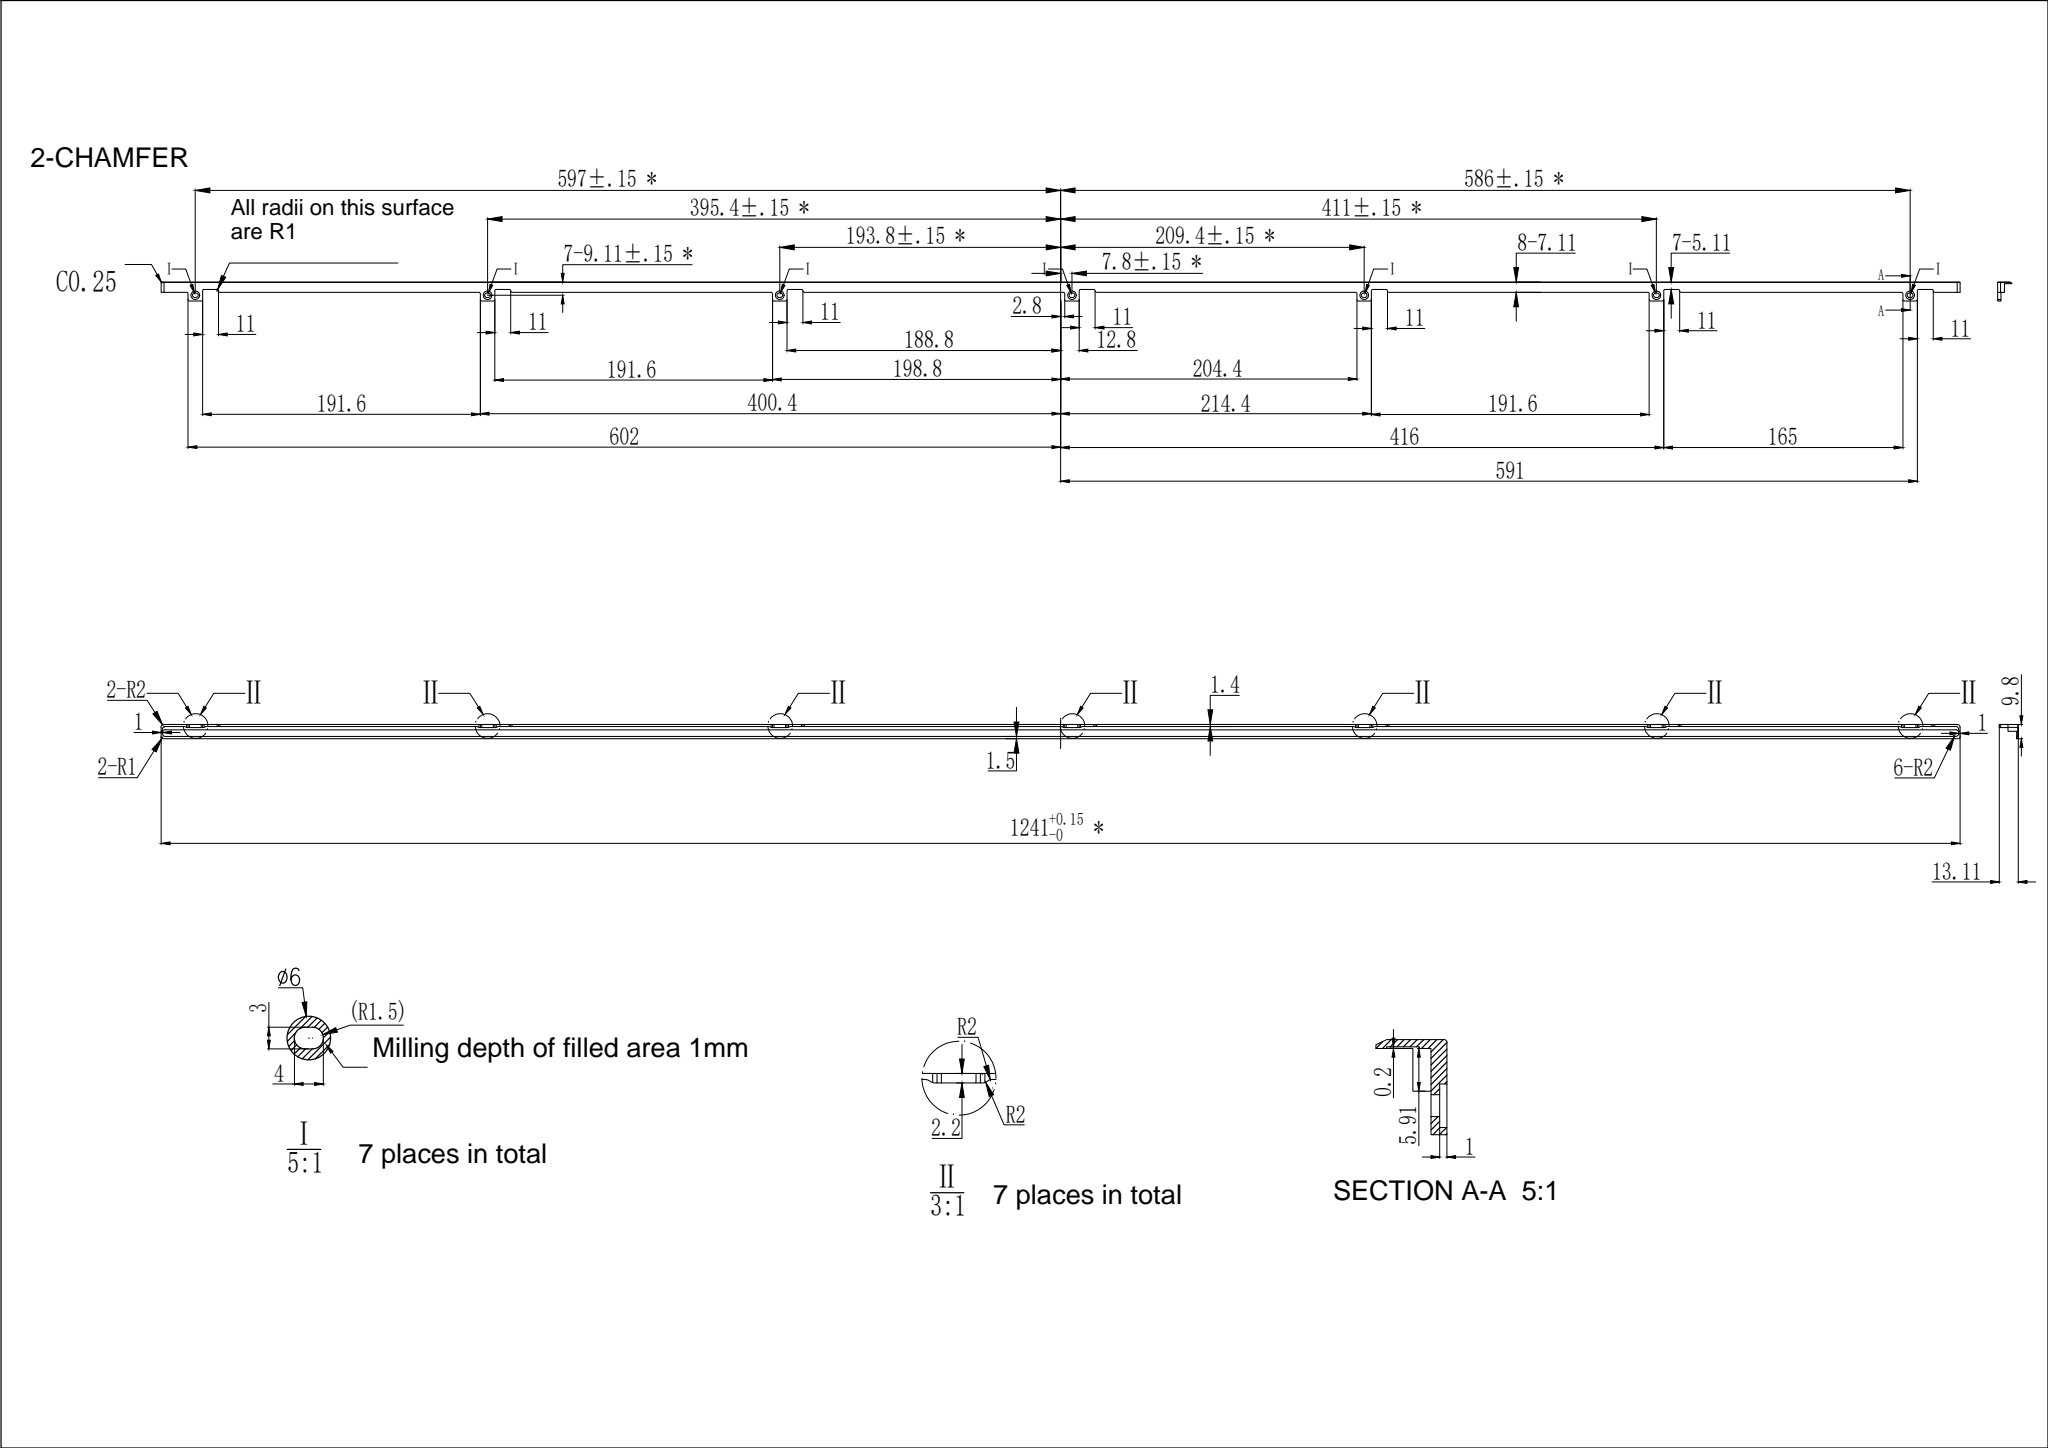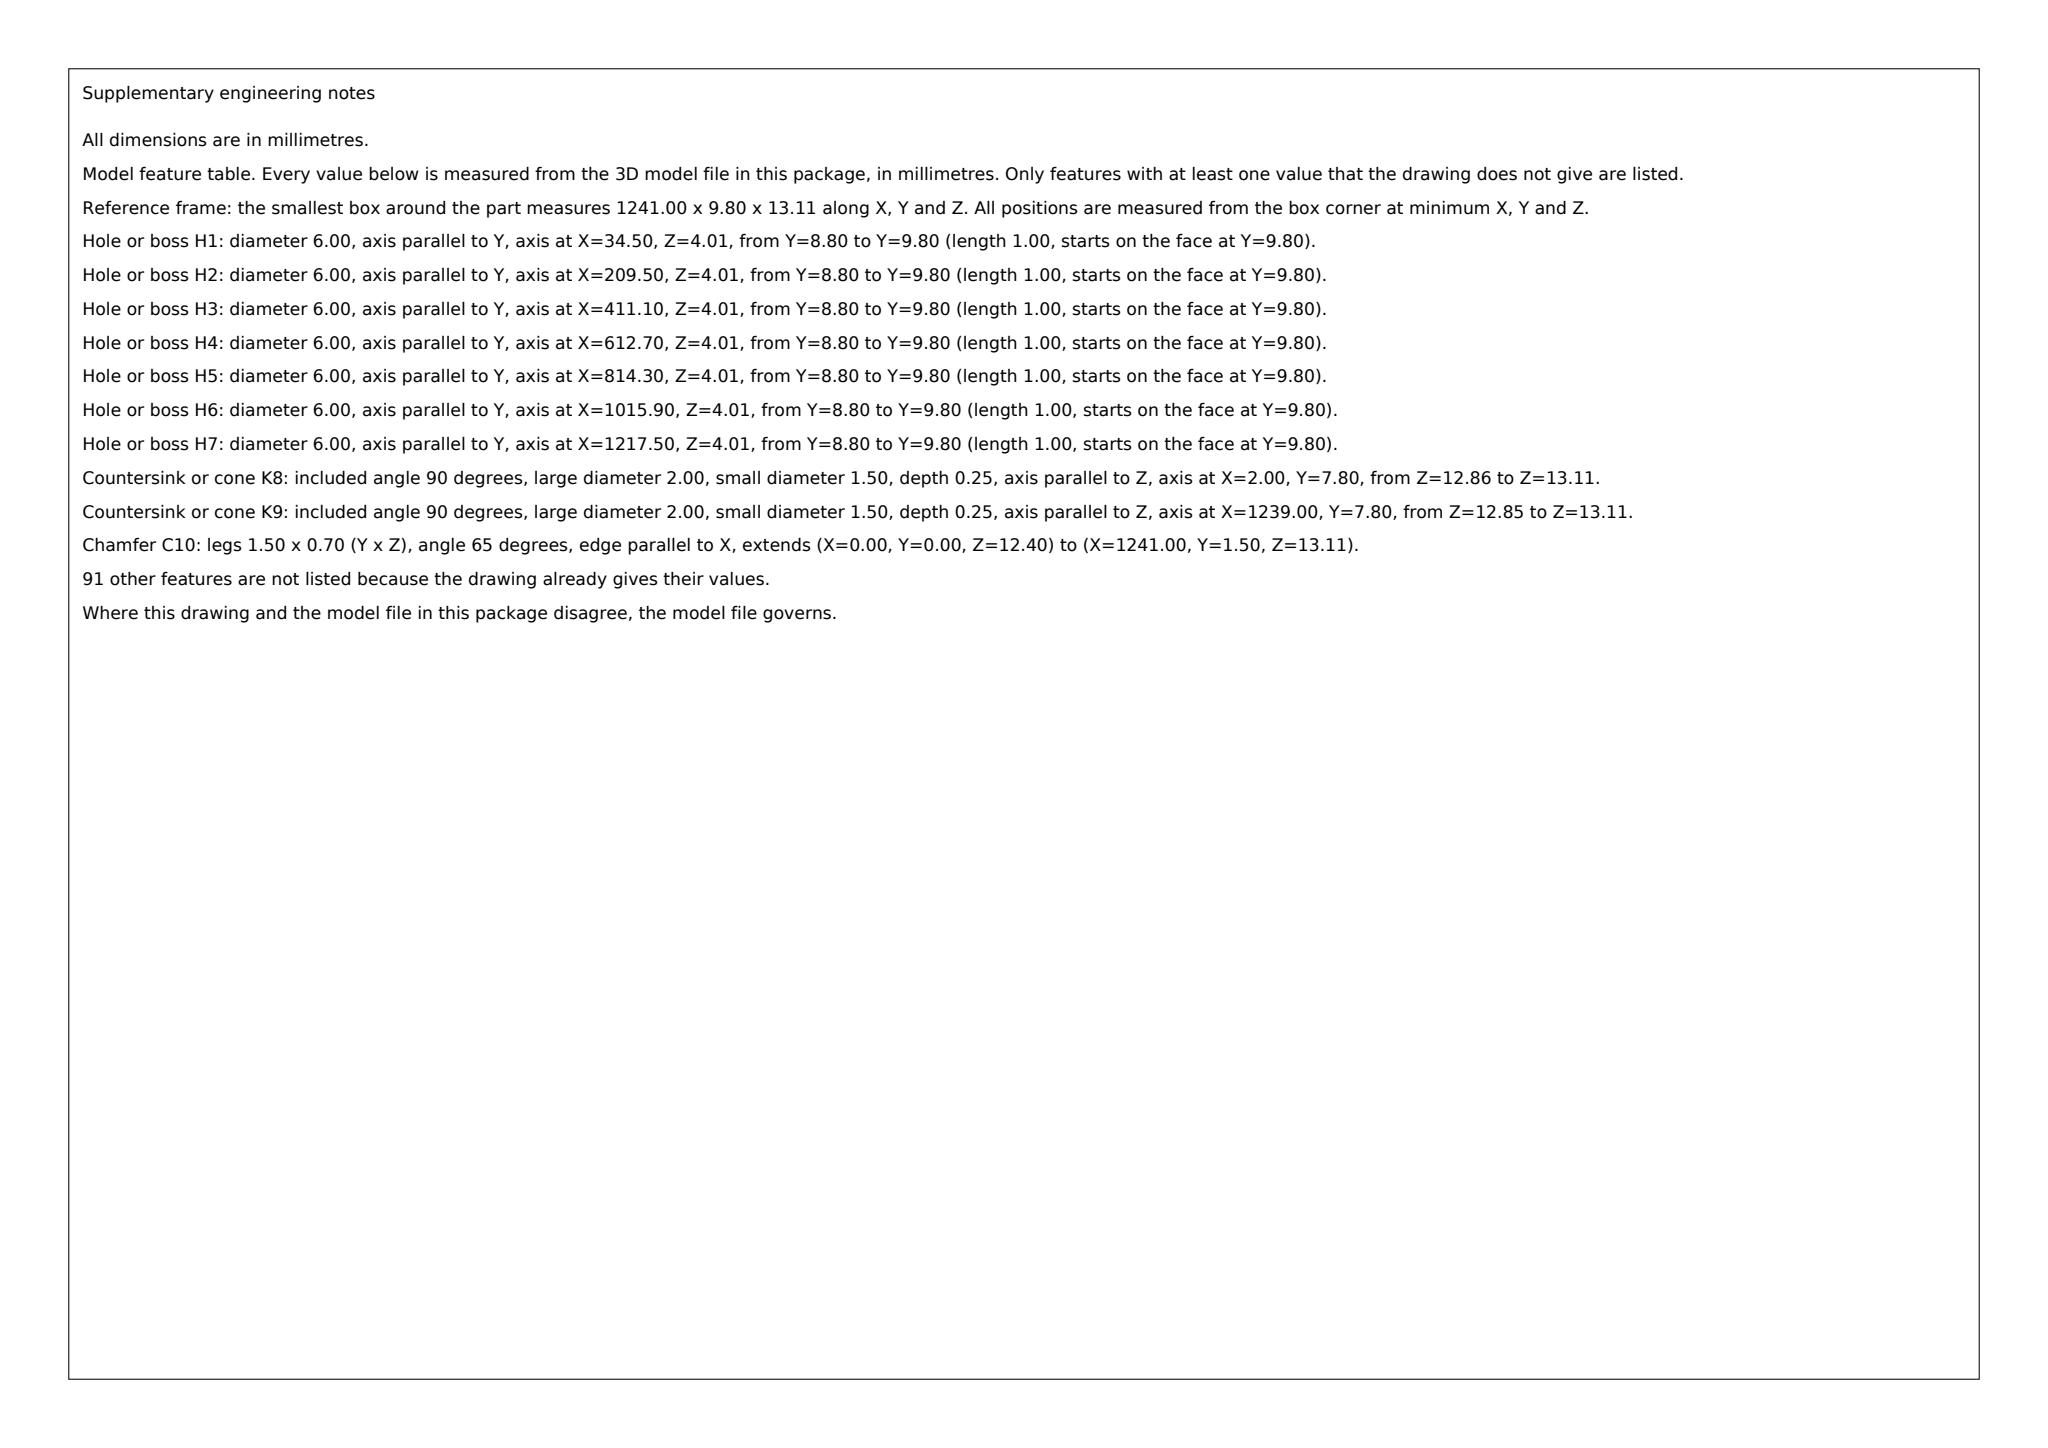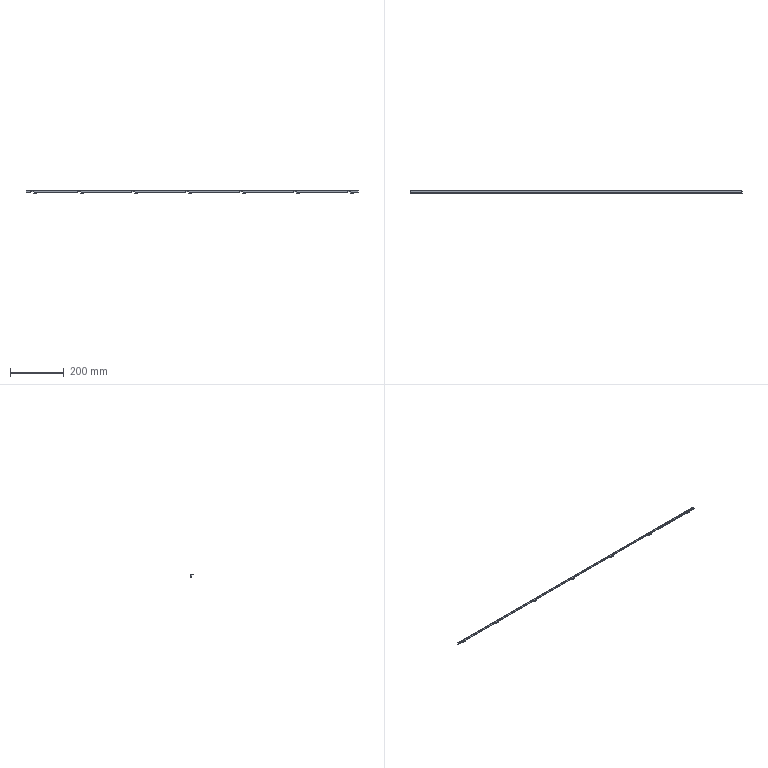Part | SolidWorks | mm | 1 solid | 194 faces | box 1241 x 9.8 x 13.11 mm | volume 23918 mm3 | cylinder 102 | plane 90 | cone 2 | commonest cylinder face diameters 2 x44 4 x30 6 x14 3 x14